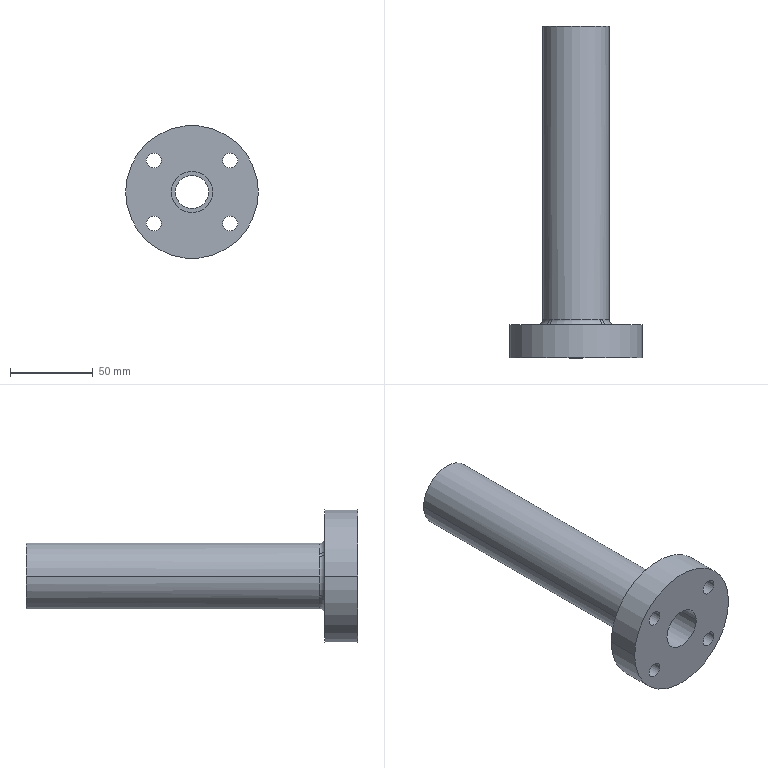Component | SolidWorks | -LimitScrewSleeve-1 | 1 solid | 41 faces | volume 227007 mm3 | cylinder 24 | plane 8 | torus 5 | spline 4 | commonest cylinder face diameters 14 x8 9 x8 25 x2 20 x2 40 x2 80 x2